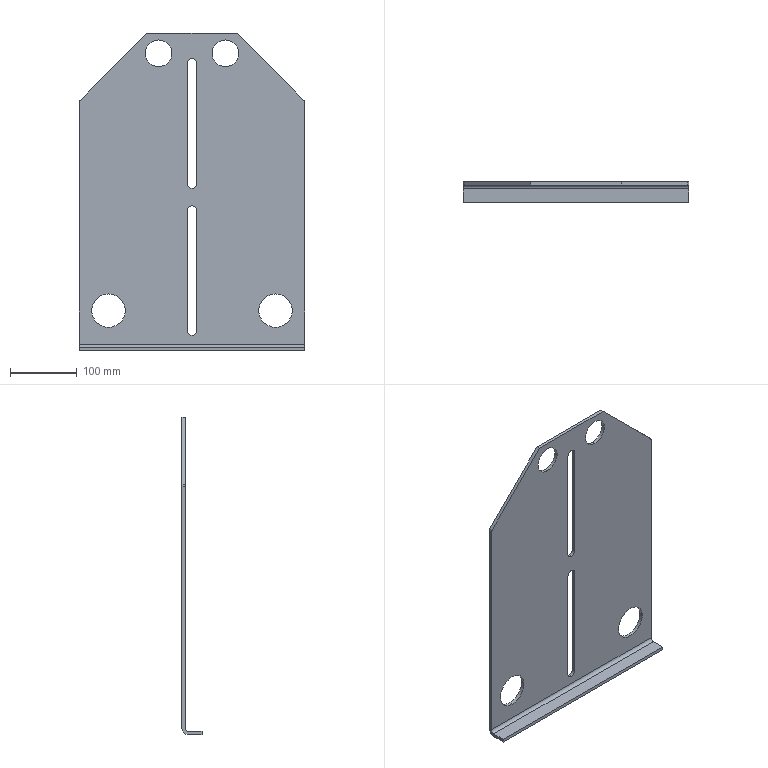Component | SolidWorks | 006TransformerBasePlate-1 | 1 solid | 32 faces | box 338 x 30 x 475 mm | volume 729103 mm3 | cylinder 18 | plane 14 | commonest cylinder face diameters 14 x6 50 x4 40 x4 10 x3 20 x1 | material Plain Carbon Steel
STEP:
#1=COLOUR_RGB('',0.7922,0.8196,0.9333);
#2=FILL_AREA_STYLE_COLOUR('',#1);
#3=FILL_AREA_STYLE('',(#2));
#4=SURFACE_STYLE_FILL_AREA(#3);
#5=SURFACE_SIDE_STYLE('',(#4));
#6=SURFACE_STYLE_USAGE(.BOTH.,#5);
#7=PRESENTATION_STYLE_ASSIGNMENT((#6));
#8=CARTESIAN_POINT('',(10.039,25.276,-15.591));
#9=VERTEX_POINT('',#8);
#10=CARTESIAN_POINT('',(10.039,25.276,-17.559));
#11=VERTEX_POINT('',#10);
#12=CARTESIAN_POINT('',(10.039,25.276,-16.575));
#13=DIRECTION('',(0.,1.,0.));
#14=DIRECTION('',(0.,0.,1.));
#15=AXIS2_PLACEMENT_3D('',#12,#13,#14);
#16=CIRCLE('',#15,0.9843);
#17=EDGE_CURVE('',#9,#11,#16,.T.);
#18=ORIENTED_EDGE('',*,*,#17,.F.);
#19=CARTESIAN_POINT('',(10.039,25.472,-15.591));
#20=VERTEX_POINT('',#19);
#21=CARTESIAN_POINT('',(10.039,24.291,-15.591));
#22=DIRECTION('',(0.,1.,0.));
#23=VECTOR('',#22,39.37);
#24=LINE('',#21,#23);
#25=EDGE_CURVE('',#9,#20,#24,.T.);
#26=ORIENTED_EDGE('',*,*,#25,.T.);
#27=CARTESIAN_POINT('',(10.039,25.472,-17.559));
#28=VERTEX_POINT('',#27);
#29=CARTESIAN_POINT('',(10.039,25.472,-16.575));
#30=DIRECTION('',(0.,1.,0.));
#31=DIRECTION('',(0.,0.,-1.));
#32=AXIS2_PLACEMENT_3D('',#29,#30,#31);
#33=CIRCLE('',#32,0.9843);
#34=EDGE_CURVE('',#20,#28,#33,.T.);
#35=ORIENTED_EDGE('',*,*,#34,.T.);
#36=CARTESIAN_POINT('',(10.039,24.291,-17.559));
#37=DIRECTION('',(0.,1.,0.));
#38=VECTOR('',#37,39.37);
#39=LINE('',#36,#38);
#40=EDGE_CURVE('',#11,#28,#39,.T.);
#41=ORIENTED_EDGE('',*,*,#40,.F.);
#42=EDGE_LOOP('',(#18,#26,#35,#41));
#43=FACE_OUTER_BOUND('',#42,.T.);
#44=CARTESIAN_POINT('',(10.039,24.291,-16.575));
#45=DIRECTION('',(0.,1.,0.));
#46=DIRECTION('',(0.,0.,-1.));
#47=AXIS2_PLACEMENT_3D('',#44,#45,#46);
#48=CYLINDRICAL_SURFACE('',#47,0.9843);
#49=ADVANCED_FACE('',(#43),#48,.F.);
#50=CARTESIAN_POINT('',(0.1969,25.276,-15.591));
#51=VERTEX_POINT('',#50);
#52=CARTESIAN_POINT('',(0.1969,25.276,-17.559));
#53=VERTEX_POINT('',#52);
#54=CARTESIAN_POINT('',(0.1969,25.276,-16.575));
#55=DIRECTION('',(0.,1.,0.));
#56=DIRECTION('',(0.,0.,1.));
#57=AXIS2_PLACEMENT_3D('',#54,#55,#56);
#58=CIRCLE('',#57,0.9843);
#59=EDGE_CURVE('',#51,#53,#58,.T.);
#60=ORIENTED_EDGE('',*,*,#59,.F.);
#61=CARTESIAN_POINT('',(0.1969,25.472,-15.591));
#62=VERTEX_POINT('',#61);
#63=CARTESIAN_POINT('',(0.1969,24.291,-15.591));
#64=DIRECTION('',(0.,1.,0.));
#65=VECTOR('',#64,39.37);
#66=LINE('',#63,#65);
#67=EDGE_CURVE('',#51,#62,#66,.T.);
#68=ORIENTED_EDGE('',*,*,#67,.T.);
#69=CARTESIAN_POINT('',(0.1969,25.472,-17.559));
#70=VERTEX_POINT('',#69);
#71=CARTESIAN_POINT('',(0.1969,25.472,-16.575));
#72=DIRECTION('',(0.,1.,0.));
#73=DIRECTION('',(0.,0.,-1.));
#74=AXIS2_PLACEMENT_3D('',#71,#72,#73);
#75=CIRCLE('',#74,0.9843);
#76=EDGE_CURVE('',#62,#70,#75,.T.);
#77=ORIENTED_EDGE('',*,*,#76,.T.);
#78=CARTESIAN_POINT('',(0.1969,24.291,-17.559));
#79=DIRECTION('',(0.,1.,0.));
#80=VECTOR('',#79,39.37);
#81=LINE('',#78,#80);
#82=EDGE_CURVE('',#53,#70,#81,.T.);
#83=ORIENTED_EDGE('',*,*,#82,.F.);
#84=EDGE_LOOP('',(#60,#68,#77,#83));
#85=FACE_OUTER_BOUND('',#84,.T.);
#86=CARTESIAN_POINT('',(0.1969,24.291,-16.575));
#87=DIRECTION('',(0.,1.,0.));
#88=DIRECTION('',(0.,0.,-1.));
#89=AXIS2_PLACEMENT_3D('',#86,#87,#88);
#90=CYLINDRICAL_SURFACE('',#89,0.9843);
#91=ADVANCED_FACE('',(#85),#90,.F.);
#92=CARTESIAN_POINT('',(7.087,25.276,-0.6299));
#93=VERTEX_POINT('',#92);
#94=CARTESIAN_POINT('',(7.087,25.276,-2.205));
#95=VERTEX_POINT('',#94);
#96=CARTESIAN_POINT('',(7.087,25.276,-1.417));
#97=DIRECTION('',(0.,1.,0.));
#98=DIRECTION('',(0.,0.,1.));
#99=AXIS2_PLACEMENT_3D('',#96,#97,#98);
#100=CIRCLE('',#99,0.7874);
#101=EDGE_CURVE('',#93,#95,#100,.T.);
#102=ORIENTED_EDGE('',*,*,#101,.F.);
#103=CARTESIAN_POINT('',(7.087,25.472,-0.6299));
#104=VERTEX_POINT('',#103);
#105=CARTESIAN_POINT('',(7.087,24.291,-0.6299));
#106=DIRECTION('',(0.,1.,0.));
#107=VECTOR('',#106,39.37);
#108=LINE('',#105,#107);
#109=EDGE_CURVE('',#93,#104,#108,.T.);
#110=ORIENTED_EDGE('',*,*,#109,.T.);
#111=CARTESIAN_POINT('',(7.087,25.472,-2.205));
#112=VERTEX_POINT('',#111);
#113=CARTESIAN_POINT('',(7.087,25.472,-1.417));
#114=DIRECTION('',(0.,1.,0.));
#115=DIRECTION('',(0.,0.,-1.));
#116=AXIS2_PLACEMENT_3D('',#113,#114,#115);
#117=CIRCLE('',#116,0.7874);
#118=EDGE_CURVE('',#104,#112,#117,.T.);
#119=ORIENTED_EDGE('',*,*,#118,.T.);
#120=CARTESIAN_POINT('',(7.087,24.291,-2.205));
#121=DIRECTION('',(0.,1.,0.));
#122=VECTOR('',#121,39.37);
#123=LINE('',#120,#122);
#124=EDGE_CURVE('',#95,#112,#123,.T.);
#125=ORIENTED_EDGE('',*,*,#124,.F.);
#126=EDGE_LOOP('',(#102,#110,#119,#125));
#127=FACE_OUTER_BOUND('',#126,.T.);
#128=CARTESIAN_POINT('',(7.087,24.291,-1.417));
#129=DIRECTION('',(0.,1.,0.));
#130=DIRECTION('',(0.,0.,-1.));
#131=AXIS2_PLACEMENT_3D('',#128,#129,#130);
#132=CYLINDRICAL_SURFACE('',#131,0.7874);
#133=ADVANCED_FACE('',(#127),#132,.F.);
#134=CARTESIAN_POINT('',(3.15,25.276,-0.6299));
#135=VERTEX_POINT('',#134);
#136=CARTESIAN_POINT('',(3.15,25.276,-2.205));
#137=VERTEX_POINT('',#136);
#138=CARTESIAN_POINT('',(3.15,25.276,-1.417));
#139=DIRECTION('',(0.,1.,0.));
#140=DIRECTION('',(0.,0.,1.));
#141=AXIS2_PLACEMENT_3D('',#138,#139,#140);
#142=CIRCLE('',#141,0.7874);
#143=EDGE_CURVE('',#135,#137,#142,.T.);
#144=ORIENTED_EDGE('',*,*,#143,.F.);
#145=CARTESIAN_POINT('',(3.15,25.472,-0.6299));
#146=VERTEX_POINT('',#145);
#147=CARTESIAN_POINT('',(3.15,24.291,-0.6299));
#148=DIRECTION('',(0.,1.,0.));
#149=VECTOR('',#148,39.37);
#150=LINE('',#147,#149);
#151=EDGE_CURVE('',#135,#146,#150,.T.);
#152=ORIENTED_EDGE('',*,*,#151,.T.);
#153=CARTESIAN_POINT('',(3.15,25.472,-2.205));
#154=VERTEX_POINT('',#153);
#155=CARTESIAN_POINT('',(3.15,25.472,-1.417));
#156=DIRECTION('',(0.,1.,0.));
#157=DIRECTION('',(0.,0.,-1.));
#158=AXIS2_PLACEMENT_3D('',#155,#156,#157);
#159=CIRCLE('',#158,0.7874);
#160=EDGE_CURVE('',#146,#154,#159,.T.);
#161=ORIENTED_EDGE('',*,*,#160,.T.);
#162=CARTESIAN_POINT('',(3.15,24.291,-2.205));
#163=DIRECTION('',(0.,1.,0.));
#164=VECTOR('',#163,39.37);
#165=LINE('',#162,#164);
#166=EDGE_CURVE('',#137,#154,#165,.T.);
#167=ORIENTED_EDGE('',*,*,#166,.F.);
#168=EDGE_LOOP('',(#144,#152,#161,#167));
#169=FACE_OUTER_BOUND('',#168,.T.);
#170=CARTESIAN_POINT('',(3.15,24.291,-1.417));
#171=DIRECTION('',(0.,1.,0.));
#172=DIRECTION('',(0.,0.,-1.));
#173=AXIS2_PLACEMENT_3D('',#170,#171,#172);
#174=CYLINDRICAL_SURFACE('',#173,0.7874);
#175=ADVANCED_FACE('',(#169),#174,.F.);
#176=CARTESIAN_POINT('',(5.118,25.276,-18.031));
#177=VERTEX_POINT('',#176);
#178=CARTESIAN_POINT('',(4.843,25.276,-17.756));
#179=VERTEX_POINT('',#178);
#180=CARTESIAN_POINT('',(5.118,25.276,-17.756));
#181=DIRECTION('',(0.,1.,0.));
#182=DIRECTION('',(0.,0.,1.));
#183=AXIS2_PLACEMENT_3D('',#180,#181,#182);
#184=CIRCLE('',#183,0.2756);
#185=EDGE_CURVE('',#177,#179,#184,.T.);
#186=ORIENTED_EDGE('',*,*,#185,.F.);
#187=CARTESIAN_POINT('',(5.118,25.472,-18.031));
#188=VERTEX_POINT('',#187);
#189=CARTESIAN_POINT('',(5.118,25.276,-18.031));
#190=DIRECTION('',(0.,1.,0.));
#191=VECTOR('',#190,39.37);
#192=LINE('',#189,#191);
#193=EDGE_CURVE('',#177,#188,#192,.T.);
#194=ORIENTED_EDGE('',*,*,#193,.T.);
#195=CARTESIAN_POINT('',(4.843,25.472,-17.756));
#196=VERTEX_POINT('',#195);
#197=CARTESIAN_POINT('',(5.118,25.472,-17.756));
#198=DIRECTION('',(0.,1.,0.));
#199=DIRECTION('',(0.,0.,-1.));
#200=AXIS2_PLACEMENT_3D('',#197,#198,#199);
#201=CIRCLE('',#200,0.2756);
#202=EDGE_CURVE('',#188,#196,#201,.T.);
#203=ORIENTED_EDGE('',*,*,#202,.T.);
#204=CARTESIAN_POINT('',(4.843,25.276,-17.756));
#205=DIRECTION('',(0.,1.,0.));
#206=VECTOR('',#205,39.37);
#207=LINE('',#204,#206);
#208=EDGE_CURVE('',#179,#196,#207,.T.);
#209=ORIENTED_EDGE('',*,*,#208,.F.);
#210=EDGE_LOOP('',(#186,#194,#203,#209));
#211=FACE_OUTER_BOUND('',#210,.T.);
#212=CARTESIAN_POINT('',(5.118,25.276,-17.756));
#213=DIRECTION('',(0.,1.,0.));
#214=DIRECTION('',(0.,0.,-1.));
#215=AXIS2_PLACEMENT_3D('',#212,#213,#214);
#216=CYLINDRICAL_SURFACE('',#215,0.2756);
#217=ADVANCED_FACE('',(#211),#216,.F.);
#218=CARTESIAN_POINT('',(5.118,25.276,-9.37));
#219=VERTEX_POINT('',#218);
#220=CARTESIAN_POINT('',(4.843,25.276,-9.094));
#221=VERTEX_POINT('',#220);
#222=CARTESIAN_POINT('',(5.118,25.276,-9.094));
#223=DIRECTION('',(0.,1.,0.));
#224=DIRECTION('',(0.,0.,1.));
#225=AXIS2_PLACEMENT_3D('',#222,#223,#224);
#226=CIRCLE('',#225,0.2756);
#227=EDGE_CURVE('',#219,#221,#226,.T.);
#228=ORIENTED_EDGE('',*,*,#227,.F.);
#229=CARTESIAN_POINT('',(5.118,25.472,-9.37));
#230=VERTEX_POINT('',#229);
#231=CARTESIAN_POINT('',(5.118,25.276,-9.37));
#232=DIRECTION('',(0.,1.,0.));
#233=VECTOR('',#232,39.37);
#234=LINE('',#231,#233);
#235=EDGE_CURVE('',#219,#230,#234,.T.);
#236=ORIENTED_EDGE('',*,*,#235,.T.);
#237=CARTESIAN_POINT('',(4.843,25.472,-9.094));
#238=VERTEX_POINT('',#237);
#239=CARTESIAN_POINT('',(5.118,25.472,-9.094));
#240=DIRECTION('',(0.,1.,0.));
#241=DIRECTION('',(0.,0.,-1.));
#242=AXIS2_PLACEMENT_3D('',#239,#240,#241);
#243=CIRCLE('',#242,0.2756);
#244=EDGE_CURVE('',#230,#238,#243,.T.);
#245=ORIENTED_EDGE('',*,*,#244,.T.);
#246=CARTESIAN_POINT('',(4.843,25.276,-9.094));
#247=DIRECTION('',(0.,1.,0.));
#248=VECTOR('',#247,39.37);
#249=LINE('',#246,#248);
#250=EDGE_CURVE('',#221,#238,#249,.T.);
#251=ORIENTED_EDGE('',*,*,#250,.F.);
#252=EDGE_LOOP('',(#228,#236,#245,#251));
#253=FACE_OUTER_BOUND('',#252,.T.);
#254=CARTESIAN_POINT('',(5.118,25.276,-9.094));
#255=DIRECTION('',(0.,1.,0.));
#256=DIRECTION('',(0.,0.,-1.));
#257=AXIS2_PLACEMENT_3D('',#254,#255,#256);
#258=CYLINDRICAL_SURFACE('',#257,0.2756);
#259=ADVANCED_FACE('',(#253),#258,.F.);
#260=CARTESIAN_POINT('',(10.039,25.276,-16.575));
#261=DIRECTION('',(0.,1.,0.));
#262=DIRECTION('',(0.,0.,1.));
#263=AXIS2_PLACEMENT_3D('',#260,#261,#262);
#264=CIRCLE('',#263,0.9843);
#265=EDGE_CURVE('',#11,#9,#264,.T.);
#266=ORIENTED_EDGE('',*,*,#265,.T.);
#267=ORIENTED_EDGE('',*,*,#17,.T.);
#268=EDGE_LOOP('',(#266,#267));
#269=FACE_BOUND('',#268,.T.);
#270=CARTESIAN_POINT('',(0.1969,25.276,-16.575));
#271=DIRECTION('',(0.,1.,0.));
#272=DIRECTION('',(0.,0.,1.));
#273=AXIS2_PLACEMENT_3D('',#270,#271,#272);
#274=CIRCLE('',#273,0.9843);
#275=EDGE_CURVE('',#53,#51,#274,.T.);
#276=ORIENTED_EDGE('',*,*,#275,.T.);
#277=ORIENTED_EDGE('',*,*,#59,.T.);
#278=EDGE_LOOP('',(#276,#277));
#279=FACE_BOUND('',#278,.T.);
#280=CARTESIAN_POINT('',(7.087,25.276,-1.417));
#281=DIRECTION('',(0.,1.,0.));
#282=DIRECTION('',(0.,0.,1.));
#283=AXIS2_PLACEMENT_3D('',#280,#281,#282);
#284=CIRCLE('',#283,0.7874);
#285=EDGE_CURVE('',#95,#93,#284,.T.);
#286=ORIENTED_EDGE('',*,*,#285,.T.);
#287=ORIENTED_EDGE('',*,*,#101,.T.);
#288=EDGE_LOOP('',(#286,#287));
#289=FACE_BOUND('',#288,.T.);
#290=CARTESIAN_POINT('',(3.15,25.276,-1.417));
#291=DIRECTION('',(0.,1.,0.));
#292=DIRECTION('',(0.,0.,1.));
#293=AXIS2_PLACEMENT_3D('',#290,#291,#292);
#294=CIRCLE('',#293,0.7874);
#295=EDGE_CURVE('',#137,#135,#294,.T.);
#296=ORIENTED_EDGE('',*,*,#295,.T.);
#297=ORIENTED_EDGE('',*,*,#143,.T.);
#298=EDGE_LOOP('',(#296,#297));
#299=FACE_BOUND('',#298,.T.);
#300=CARTESIAN_POINT('',(4.843,25.276,-10.669));
#301=VERTEX_POINT('',#300);
#302=CARTESIAN_POINT('',(5.394,25.276,-10.669));
#303=VERTEX_POINT('',#302);
#304=CARTESIAN_POINT('',(5.118,25.276,-10.669));
#305=DIRECTION('',(0.,1.,0.));
#306=DIRECTION('',(0.,0.,1.));
#307=AXIS2_PLACEMENT_3D('',#304,#305,#306);
#308=CIRCLE('',#307,0.2756);
#309=EDGE_CURVE('',#301,#303,#308,.T.);
#310=ORIENTED_EDGE('',*,*,#309,.T.);
#311=CARTESIAN_POINT('',(5.394,25.276,-17.756));
#312=VERTEX_POINT('',#311);
#313=CARTESIAN_POINT('',(5.394,25.276,-10.669));
#314=DIRECTION('',(0.,0.,-1.));
#315=VECTOR('',#314,39.37);
#316=LINE('',#313,#315);
#317=EDGE_CURVE('',#303,#312,#316,.T.);
#318=ORIENTED_EDGE('',*,*,#317,.T.);
#319=CARTESIAN_POINT('',(5.118,25.276,-17.756));
#320=DIRECTION('',(0.,1.,0.));
#321=DIRECTION('',(0.,0.,1.));
#322=AXIS2_PLACEMENT_3D('',#319,#320,#321);
#323=CIRCLE('',#322,0.2756);
#324=EDGE_CURVE('',#312,#177,#323,.T.);
#325=ORIENTED_EDGE('',*,*,#324,.T.);
#326=ORIENTED_EDGE('',*,*,#185,.T.);
#327=CARTESIAN_POINT('',(4.843,25.276,-10.669));
#328=DIRECTION('',(-0.,0.,1.));
#329=VECTOR('',#328,39.37);
#330=LINE('',#327,#329);
#331=EDGE_CURVE('',#179,#301,#330,.T.);
#332=ORIENTED_EDGE('',*,*,#331,.T.);
#333=EDGE_LOOP('',(#310,#318,#325,#326,#332));
#334=FACE_BOUND('',#333,.T.);
#335=CARTESIAN_POINT('',(4.843,25.276,-2.008));
#336=VERTEX_POINT('',#335);
#337=CARTESIAN_POINT('',(5.394,25.276,-2.008));
#338=VERTEX_POINT('',#337);
#339=CARTESIAN_POINT('',(5.118,25.276,-2.008));
#340=DIRECTION('',(0.,1.,0.));
#341=DIRECTION('',(0.,0.,1.));
#342=AXIS2_PLACEMENT_3D('',#339,#340,#341);
#343=CIRCLE('',#342,0.2756);
#344=EDGE_CURVE('',#336,#338,#343,.T.);
#345=ORIENTED_EDGE('',*,*,#344,.T.);
#346=CARTESIAN_POINT('',(5.394,25.276,-9.094));
#347=VERTEX_POINT('',#346);
#348=CARTESIAN_POINT('',(5.394,25.276,-2.008));
#349=DIRECTION('',(0.,0.,-1.));
#350=VECTOR('',#349,39.37);
#351=LINE('',#348,#350);
#352=EDGE_CURVE('',#338,#347,#351,.T.);
#353=ORIENTED_EDGE('',*,*,#352,.T.);
#354=CARTESIAN_POINT('',(5.118,25.276,-9.094));
#355=DIRECTION('',(0.,1.,0.));
#356=DIRECTION('',(0.,0.,1.));
#357=AXIS2_PLACEMENT_3D('',#354,#355,#356);
#358=CIRCLE('',#357,0.2756);
#359=EDGE_CURVE('',#347,#219,#358,.T.);
#360=ORIENTED_EDGE('',*,*,#359,.T.);
#361=ORIENTED_EDGE('',*,*,#227,.T.);
#362=CARTESIAN_POINT('',(4.843,25.276,-2.008));
#363=DIRECTION('',(0.,0.,1.));
#364=VECTOR('',#363,39.37);
#365=LINE('',#362,#364);
#366=EDGE_CURVE('',#221,#336,#365,.T.);
#367=ORIENTED_EDGE('',*,*,#366,.T.);
#368=EDGE_LOOP('',(#345,#353,#360,#361,#367));
#369=FACE_BOUND('',#368,.T.);
#370=CARTESIAN_POINT('',(-1.535,25.276,-18.543));
#371=VERTEX_POINT('',#370);
#372=CARTESIAN_POINT('',(-1.535,25.276,-4.314));
#373=VERTEX_POINT('',#372);
#374=CARTESIAN_POINT('',(-1.535,25.276,-4.232));
#375=DIRECTION('',(-0.,0.,1.));
#376=VECTOR('',#375,39.37);
#377=LINE('',#374,#376);
#378=EDGE_CURVE('',#371,#373,#377,.T.);
#379=ORIENTED_EDGE('',*,*,#378,.F.);
#380=CARTESIAN_POINT('',(11.772,25.276,-18.543));
#381=VERTEX_POINT('',#380);
#382=CARTESIAN_POINT('',(11.772,25.276,-18.543));
#383=DIRECTION('',(1.,0.,0.));
#384=VECTOR('',#383,39.37);
#385=LINE('',#382,#384);
#386=EDGE_CURVE('',#371,#381,#385,.T.);
#387=ORIENTED_EDGE('',*,*,#386,.T.);
#388=CARTESIAN_POINT('',(11.772,25.276,-4.314));
#389=VERTEX_POINT('',#388);
#390=CARTESIAN_POINT('',(11.772,25.276,-4.232));
#391=DIRECTION('',(-0.,0.,-1.));
#392=VECTOR('',#391,39.37);
#393=LINE('',#390,#392);
#394=EDGE_CURVE('',#389,#381,#393,.T.);
#395=ORIENTED_EDGE('',*,*,#394,.F.);
#396=CARTESIAN_POINT('',(11.714,25.276,-4.175));
#397=VERTEX_POINT('',#396);
#398=CARTESIAN_POINT('',(11.575,25.276,-4.314));
#399=DIRECTION('',(0.,-1.,0.));
#400=DIRECTION('',(0.,0.,1.));
#401=AXIS2_PLACEMENT_3D('',#398,#399,#400);
#402=CIRCLE('',#401,0.1969);
#403=EDGE_CURVE('',#389,#397,#402,.T.);
#404=ORIENTED_EDGE('',*,*,#403,.T.);
#405=CARTESIAN_POINT('',(7.776,25.276,-0.2362));
#406=VERTEX_POINT('',#405);
#407=CARTESIAN_POINT('',(11.772,25.276,-4.232));
#408=DIRECTION('',(0.7071,0.,-0.7071));
#409=VECTOR('',#408,39.37);
#410=LINE('',#407,#409);
#411=EDGE_CURVE('',#406,#397,#410,.T.);
#412=ORIENTED_EDGE('',*,*,#411,.F.);
#413=CARTESIAN_POINT('',(2.461,25.276,-0.2362));
#414=VERTEX_POINT('',#413);
#415=CARTESIAN_POINT('',(7.776,25.276,-0.2362));
#416=DIRECTION('',(1.,0.,0.));
#417=VECTOR('',#416,39.37);
#418=LINE('',#415,#417);
#419=EDGE_CURVE('',#414,#406,#418,.T.);
#420=ORIENTED_EDGE('',*,*,#419,.F.);
#421=CARTESIAN_POINT('',(-1.478,25.276,-4.175));
#422=VERTEX_POINT('',#421);
#423=CARTESIAN_POINT('',(-1.535,25.276,-4.232));
#424=DIRECTION('',(0.7071,0.,0.7071));
#425=VECTOR('',#424,39.37);
#426=LINE('',#423,#425);
#427=EDGE_CURVE('',#422,#414,#426,.T.);
#428=ORIENTED_EDGE('',*,*,#427,.F.);
#429=CARTESIAN_POINT('',(-1.339,25.276,-4.314));
#430=DIRECTION('',(0.,-1.,0.));
#431=DIRECTION('',(0.,0.,1.));
#432=AXIS2_PLACEMENT_3D('',#429,#430,#431);
#433=CIRCLE('',#432,0.1969);
#434=EDGE_CURVE('',#422,#373,#433,.T.);
#435=ORIENTED_EDGE('',*,*,#434,.T.);
#436=EDGE_LOOP('',(#379,#387,#395,#404,#412,#420,#428,#435));
#437=FACE_OUTER_BOUND('',#436,.T.);
#438=CARTESIAN_POINT('',(-1.535,25.276,-18.937));
#439=DIRECTION('',(0.,-1.,0.));
#440=DIRECTION('',(0.,0.,1.));
#441=AXIS2_PLACEMENT_3D('',#438,#439,#440);
#442=PLANE('',#441);
#443=ADVANCED_FACE('',(#269,#279,#289,#299,#334,#369,#437),#442,.T.);
#444=CARTESIAN_POINT('',(-1.535,25.079,-18.937));
#445=VERTEX_POINT('',#444);
#446=CARTESIAN_POINT('',(-1.535,24.291,-18.937));
#447=VERTEX_POINT('',#446);
#448=CARTESIAN_POINT('',(-1.535,25.472,-18.937));
#449=DIRECTION('',(0.,-1.,0.));
#450=VECTOR('',#449,39.37);
#451=LINE('',#448,#450);
#452=EDGE_CURVE('',#445,#447,#451,.T.);
#453=ORIENTED_EDGE('',*,*,#452,.F.);
#454=CARTESIAN_POINT('',(11.772,25.079,-18.937));
#455=VERTEX_POINT('',#454);
#456=CARTESIAN_POINT('',(11.772,25.079,-18.937));
#457=DIRECTION('',(1.,0.,0.));
#458=VECTOR('',#457,39.37);
#459=LINE('',#456,#458);
#460=EDGE_CURVE('',#445,#455,#459,.T.);
#461=ORIENTED_EDGE('',*,*,#460,.T.);
#462=CARTESIAN_POINT('',(11.772,24.291,-18.937));
#463=VERTEX_POINT('',#462);
#464=CARTESIAN_POINT('',(11.772,25.472,-18.937));
#465=DIRECTION('',(0.,-1.,0.));
#466=VECTOR('',#465,39.37);
#467=LINE('',#464,#466);
#468=EDGE_CURVE('',#455,#463,#467,.T.);
#469=ORIENTED_EDGE('',*,*,#468,.T.);
#470=CARTESIAN_POINT('',(-2.539,24.291,-18.937));
#471=DIRECTION('',(1.,0.,0.));
#472=VECTOR('',#471,39.37);
#473=LINE('',#470,#472);
#474=EDGE_CURVE('',#447,#463,#473,.T.);
#475=ORIENTED_EDGE('',*,*,#474,.F.);
#476=EDGE_LOOP('',(#453,#461,#469,#475));
#477=FACE_OUTER_BOUND('',#476,.T.);
#478=CARTESIAN_POINT('',(11.772,25.472,-18.937));
#479=DIRECTION('',(0.,0.,1.));
#480=DIRECTION('',(0.,1.,0.));
#481=AXIS2_PLACEMENT_3D('',#478,#479,#480);
#482=PLANE('',#481);
#483=ADVANCED_FACE('',(#477),#482,.F.);
#484=CARTESIAN_POINT('',(-1.535,25.472,-18.543));
#485=VERTEX_POINT('',#484);
#486=CARTESIAN_POINT('',(-1.535,25.472,-4.314));
#487=VERTEX_POINT('',#486);
#488=CARTESIAN_POINT('',(-1.535,25.472,-4.232));
#489=DIRECTION('',(-0.,0.,1.));
#490=VECTOR('',#489,39.37);
#491=LINE('',#488,#490);
#492=EDGE_CURVE('',#485,#487,#491,.T.);
#493=ORIENTED_EDGE('',*,*,#492,.F.);
#494=CARTESIAN_POINT('',(-1.535,25.079,-18.543));
#495=DIRECTION('',(-1.,0.,-0.));
#496=DIRECTION('',(0.,0.,-1.));
#497=AXIS2_PLACEMENT_3D('',#494,#495,#496);
#498=CIRCLE('',#497,0.3937);
#499=EDGE_CURVE('',#485,#445,#498,.T.);
#500=ORIENTED_EDGE('',*,*,#499,.T.);
#501=ORIENTED_EDGE('',*,*,#452,.T.);
#502=CARTESIAN_POINT('',(-1.535,24.291,-18.74));
#503=VERTEX_POINT('',#502);
#504=CARTESIAN_POINT('',(-1.535,24.291,-18.74));
#505=DIRECTION('',(-0.,0.,1.));
#506=VECTOR('',#505,39.37);
#507=LINE('',#504,#506);
#508=EDGE_CURVE('',#447,#503,#507,.T.);
#509=ORIENTED_EDGE('',*,*,#508,.T.);
#510=CARTESIAN_POINT('',(-1.535,25.079,-18.74));
#511=VERTEX_POINT('',#510);
#512=CARTESIAN_POINT('',(-1.535,25.276,-18.74));
#513=DIRECTION('',(-0.,1.,0.));
#514=VECTOR('',#513,39.37);
#515=LINE('',#512,#514);
#516=EDGE_CURVE('',#503,#511,#515,.T.);
#517=ORIENTED_EDGE('',*,*,#516,.T.);
#518=CARTESIAN_POINT('',(-1.535,25.079,-18.543));
#519=DIRECTION('',(1.,0.,0.));
#520=DIRECTION('',(0.,0.,-1.));
#521=AXIS2_PLACEMENT_3D('',#518,#519,#520);
#522=CIRCLE('',#521,0.1969);
#523=EDGE_CURVE('',#511,#371,#522,.T.);
#524=ORIENTED_EDGE('',*,*,#523,.T.);
#525=ORIENTED_EDGE('',*,*,#378,.T.);
#526=CARTESIAN_POINT('',(-1.535,25.472,-4.314));
#527=DIRECTION('',(0.,1.,0.));
#528=VECTOR('',#527,39.37);
#529=LINE('',#526,#528);
#530=EDGE_CURVE('',#373,#487,#529,.T.);
#531=ORIENTED_EDGE('',*,*,#530,.T.);
#532=EDGE_LOOP('',(#493,#500,#501,#509,#517,#524,#525,#531));
#533=FACE_OUTER_BOUND('',#532,.T.);
#534=CARTESIAN_POINT('',(-1.535,25.472,-4.232));
#535=DIRECTION('',(1.,0.,0.));
#536=DIRECTION('',(0.,0.,-1.));
#537=AXIS2_PLACEMENT_3D('',#534,#535,#536);
#538=PLANE('',#537);
#539=ADVANCED_FACE('',(#533),#538,.F.);
#540=CARTESIAN_POINT('',(-1.478,25.472,-4.175));
#541=VERTEX_POINT('',#540);
#542=CARTESIAN_POINT('',(2.461,25.472,-0.2362));
#543=VERTEX_POINT('',#542);
#544=CARTESIAN_POINT('',(-1.535,25.472,-4.232));
#545=DIRECTION('',(0.7071,0.,0.7071));
#546=VECTOR('',#545,39.37);
#547=LINE('',#544,#546);
#548=EDGE_CURVE('',#541,#543,#547,.T.);
#549=ORIENTED_EDGE('',*,*,#548,.F.);
#550=CARTESIAN_POINT('',(-1.478,25.472,-4.175));
#551=DIRECTION('',(0.,-1.,0.));
#552=VECTOR('',#551,39.37);
#553=LINE('',#550,#552);
#554=EDGE_CURVE('',#541,#422,#553,.T.);
#555=ORIENTED_EDGE('',*,*,#554,.T.);
#556=ORIENTED_EDGE('',*,*,#427,.T.);
#557=CARTESIAN_POINT('',(2.461,25.472,-0.2362));
#558=DIRECTION('',(0.,-1.,0.));
#559=VECTOR('',#558,39.37);
#560=LINE('',#557,#559);
#561=EDGE_CURVE('',#543,#414,#560,.T.);
#562=ORIENTED_EDGE('',*,*,#561,.F.);
#563=EDGE_LOOP('',(#549,#555,#556,#562));
#564=FACE_OUTER_BOUND('',#563,.T.);
#565=CARTESIAN_POINT('',(-1.535,25.472,-4.232));
#566=DIRECTION('',(0.7071,0.,-0.7071));
#567=DIRECTION('',(-0.7071,0.,-0.7071));
#568=AXIS2_PLACEMENT_3D('',#565,#566,#567);
#569=PLANE('',#568);
#570=ADVANCED_FACE('',(#564),#569,.F.);
#571=ORIENTED_EDGE('',*,*,#419,.T.);
#572=CARTESIAN_POINT('',(7.776,25.472,-0.2362));
#573=VERTEX_POINT('',#572);
#574=CARTESIAN_POINT('',(7.776,25.472,-0.2362));
#575=DIRECTION('',(0.,-1.,0.));
#576=VECTOR('',#575,39.37);
#577=LINE('',#574,#576);
#578=EDGE_CURVE('',#573,#406,#577,.T.);
#579=ORIENTED_EDGE('',*,*,#578,.F.);
#580=CARTESIAN_POINT('',(7.776,25.472,-0.2362));
#581=DIRECTION('',(1.,0.,0.));
#582=VECTOR('',#581,39.37);
#583=LINE('',#580,#582);
#584=EDGE_CURVE('',#543,#573,#583,.T.);
#585=ORIENTED_EDGE('',*,*,#584,.F.);
#586=ORIENTED_EDGE('',*,*,#561,.T.);
#587=EDGE_LOOP('',(#571,#579,#585,#586));
#588=FACE_OUTER_BOUND('',#587,.T.);
#589=CARTESIAN_POINT('',(7.776,25.472,-0.2362));
#590=DIRECTION('',(0.,0.,-1.));
#591=DIRECTION('',(0.,-1.,0.));
#592=AXIS2_PLACEMENT_3D('',#589,#590,#591);
#593=PLANE('',#592);
#594=ADVANCED_FACE('',(#588),#593,.F.);
#595=ORIENTED_EDGE('',*,*,#411,.T.);
#596=CARTESIAN_POINT('',(11.714,25.472,-4.175));
#597=VERTEX_POINT('',#596);
#598=CARTESIAN_POINT('',(11.714,25.472,-4.175));
#599=DIRECTION('',(0.,1.,0.));
#600=VECTOR('',#599,39.37);
#601=LINE('',#598,#600);
#602=EDGE_CURVE('',#397,#597,#601,.T.);
#603=ORIENTED_EDGE('',*,*,#602,.T.);
#604=CARTESIAN_POINT('',(11.772,25.472,-4.232));
#605=DIRECTION('',(0.7071,0.,-0.7071));
#606=VECTOR('',#605,39.37);
#607=LINE('',#604,#606);
#608=EDGE_CURVE('',#573,#597,#607,.T.);
#609=ORIENTED_EDGE('',*,*,#608,.F.);
#610=ORIENTED_EDGE('',*,*,#578,.T.);
#611=EDGE_LOOP('',(#595,#603,#609,#610));
#612=FACE_OUTER_BOUND('',#611,.T.);
#613=CARTESIAN_POINT('',(11.772,25.472,-4.232));
#614=DIRECTION('',(-0.7071,0.,-0.7071));
#615=DIRECTION('',(-0.7071,0.,0.7071));
#616=AXIS2_PLACEMENT_3D('',#613,#614,#615);
#617=PLANE('',#616);
#618=ADVANCED_FACE('',(#612),#617,.F.);
#619=ORIENTED_EDGE('',*,*,#468,.F.);
#620=CARTESIAN_POINT('',(11.772,25.472,-18.543));
#621=VERTEX_POINT('',#620);
#622=CARTESIAN_POINT('',(11.772,25.079,-18.543));
#623=DIRECTION('',(1.,0.,-0.));
#624=DIRECTION('',(0.,0.,1.));
#625=AXIS2_PLACEMENT_3D('',#622,#623,#624);
#626=CIRCLE('',#625,0.3937);
#627=EDGE_CURVE('',#455,#621,#626,.T.);
#628=ORIENTED_EDGE('',*,*,#627,.T.);
#629=CARTESIAN_POINT('',(11.772,25.472,-4.314));
#630=VERTEX_POINT('',#629);
#631=CARTESIAN_POINT('',(11.772,25.472,-4.232));
#632=DIRECTION('',(-0.,0.,-1.));
#633=VECTOR('',#632,39.37);
#634=LINE('',#631,#633);
#635=EDGE_CURVE('',#630,#621,#634,.T.);
#636=ORIENTED_EDGE('',*,*,#635,.F.);
#637=CARTESIAN_POINT('',(11.772,25.472,-4.314));
#638=DIRECTION('',(0.,-1.,0.));
#639=VECTOR('',#638,39.37);
#640=LINE('',#637,#639);
#641=EDGE_CURVE('',#630,#389,#640,.T.);
#642=ORIENTED_EDGE('',*,*,#641,.T.);
#643=ORIENTED_EDGE('',*,*,#394,.T.);
#644=CARTESIAN_POINT('',(11.772,25.079,-18.74));
#645=VERTEX_POINT('',#644);
#646=CARTESIAN_POINT('',(11.772,25.079,-18.543));
#647=DIRECTION('',(-1.,0.,0.));
#648=DIRECTION('',(0.,0.,1.));
#649=AXIS2_PLACEMENT_3D('',#646,#647,#648);
#650=CIRCLE('',#649,0.1969);
#651=EDGE_CURVE('',#381,#645,#650,.T.);
#652=ORIENTED_EDGE('',*,*,#651,.T.);
#653=CARTESIAN_POINT('',(11.772,24.291,-18.74));
#654=VERTEX_POINT('',#653);
#655=CARTESIAN_POINT('',(11.772,25.276,-18.74));
#656=DIRECTION('',(0.,-1.,-0.));
#657=VECTOR('',#656,39.37);
#658=LINE('',#655,#657);
#659=EDGE_CURVE('',#645,#654,#658,.T.);
#660=ORIENTED_EDGE('',*,*,#659,.T.);
#661=CARTESIAN_POINT('',(11.772,24.291,-18.74));
#662=DIRECTION('',(0.,0.,-1.));
#663=VECTOR('',#662,39.37);
#664=LINE('',#661,#663);
#665=EDGE_CURVE('',#654,#463,#664,.T.);
#666=ORIENTED_EDGE('',*,*,#665,.T.);
#667=EDGE_LOOP('',(#619,#628,#636,#642,#643,#652,#660,#666));
#668=FACE_OUTER_BOUND('',#667,.T.);
#669=CARTESIAN_POINT('',(11.772,25.472,-4.232));
#670=DIRECTION('',(-1.,0.,0.));
#671=DIRECTION('',(0.,0.,1.));
#672=AXIS2_PLACEMENT_3D('',#669,#670,#671);
#673=PLANE('',#672);
#674=ADVANCED_FACE('',(#668),#673,.F.);
#675=CARTESIAN_POINT('',(10.039,25.472,-16.575));
#676=DIRECTION('',(0.,1.,0.));
#677=DIRECTION('',(0.,0.,-1.));
#678=AXIS2_PLACEMENT_3D('',#675,#676,#677);
#679=CIRCLE('',#678,0.9843);
#680=EDGE_CURVE('',#28,#20,#679,.T.);
#681=ORIENTED_EDGE('',*,*,#680,.F.);
#682=ORIENTED_EDGE('',*,*,#34,.F.);
#683=EDGE_LOOP('',(#681,#682));
#684=FACE_BOUND('',#683,.T.);
#685=CARTESIAN_POINT('',(0.1969,25.472,-16.575));
#686=DIRECTION('',(0.,1.,0.));
#687=DIRECTION('',(0.,0.,-1.));
#688=AXIS2_PLACEMENT_3D('',#685,#686,#687);
#689=CIRCLE('',#688,0.9843);
#690=EDGE_CURVE('',#70,#62,#689,.T.);
#691=ORIENTED_EDGE('',*,*,#690,.F.);
#692=ORIENTED_EDGE('',*,*,#76,.F.);
#693=EDGE_LOOP('',(#691,#692));
#694=FACE_BOUND('',#693,.T.);
#695=CARTESIAN_POINT('',(7.087,25.472,-1.417));
#696=DIRECTION('',(0.,1.,0.));
#697=DIRECTION('',(0.,0.,-1.));
#698=AXIS2_PLACEMENT_3D('',#695,#696,#697);
#699=CIRCLE('',#698,0.7874);
#700=EDGE_CURVE('',#112,#104,#699,.T.);
#701=ORIENTED_EDGE('',*,*,#700,.F.);
#702=ORIENTED_EDGE('',*,*,#118,.F.);
#703=EDGE_LOOP('',(#701,#702));
#704=FACE_BOUND('',#703,.T.);
#705=CARTESIAN_POINT('',(3.15,25.472,-1.417));
#706=DIRECTION('',(0.,1.,0.));
#707=DIRECTION('',(0.,0.,-1.));
#708=AXIS2_PLACEMENT_3D('',#705,#706,#707);
#709=CIRCLE('',#708,0.7874);
#710=EDGE_CURVE('',#154,#146,#709,.T.);
#711=ORIENTED_EDGE('',*,*,#710,.F.);
#712=ORIENTED_EDGE('',*,*,#160,.F.);
#713=EDGE_LOOP('',(#711,#712));
#714=FACE_BOUND('',#713,.T.);
#715=CARTESIAN_POINT('',(5.394,25.472,-10.669));
#716=VERTEX_POINT('',#715);
#717=CARTESIAN_POINT('',(5.394,25.472,-17.756));
#718=VERTEX_POINT('',#717);
#719=CARTESIAN_POINT('',(5.394,25.472,-10.669));
#720=DIRECTION('',(0.,0.,-1.));
#721=VECTOR('',#720,39.37);
#722=LINE('',#719,#721);
#723=EDGE_CURVE('',#716,#718,#722,.T.);
#724=ORIENTED_EDGE('',*,*,#723,.F.);
#725=CARTESIAN_POINT('',(4.843,25.472,-10.669));
#726=VERTEX_POINT('',#725);
#727=CARTESIAN_POINT('',(5.118,25.472,-10.669));
#728=DIRECTION('',(0.,1.,0.));
#729=DIRECTION('',(0.,0.,-1.));
#730=AXIS2_PLACEMENT_3D('',#727,#728,#729);
#731=CIRCLE('',#730,0.2756);
#732=EDGE_CURVE('',#726,#716,#731,.T.);
#733=ORIENTED_EDGE('',*,*,#732,.F.);
#734=CARTESIAN_POINT('',(4.843,25.472,-10.669));
#735=DIRECTION('',(-0.,0.,1.));
#736=VECTOR('',#735,39.37);
#737=LINE('',#734,#736);
#738=EDGE_CURVE('',#196,#726,#737,.T.);
#739=ORIENTED_EDGE('',*,*,#738,.F.);
#740=ORIENTED_EDGE('',*,*,#202,.F.);
#741=CARTESIAN_POINT('',(5.118,25.472,-17.756));
#742=DIRECTION('',(0.,1.,0.));
#743=DIRECTION('',(0.,0.,-1.));
#744=AXIS2_PLACEMENT_3D('',#741,#742,#743);
#745=CIRCLE('',#744,0.2756);
#746=EDGE_CURVE('',#718,#188,#745,.T.);
#747=ORIENTED_EDGE('',*,*,#746,.F.);
#748=EDGE_LOOP('',(#724,#733,#739,#740,#747));
#749=FACE_BOUND('',#748,.T.);
#750=CARTESIAN_POINT('',(5.394,25.472,-2.008));
#751=VERTEX_POINT('',#750);
#752=CARTESIAN_POINT('',(5.394,25.472,-9.094));
#753=VERTEX_POINT('',#752);
#754=CARTESIAN_POINT('',(5.394,25.472,-2.008));
#755=DIRECTION('',(0.,0.,-1.));
#756=VECTOR('',#755,39.37);
#757=LINE('',#754,#756);
#758=EDGE_CURVE('',#751,#753,#757,.T.);
#759=ORIENTED_EDGE('',*,*,#758,.F.);
#760=CARTESIAN_POINT('',(4.843,25.472,-2.008));
#761=VERTEX_POINT('',#760);
#762=CARTESIAN_POINT('',(5.118,25.472,-2.008));
#763=DIRECTION('',(0.,1.,0.));
#764=DIRECTION('',(0.,0.,-1.));
#765=AXIS2_PLACEMENT_3D('',#762,#763,#764);
#766=CIRCLE('',#765,0.2756);
#767=EDGE_CURVE('',#761,#751,#766,.T.);
#768=ORIENTED_EDGE('',*,*,#767,.F.);
#769=CARTESIAN_POINT('',(4.843,25.472,-2.008));
#770=DIRECTION('',(0.,0.,1.));
#771=VECTOR('',#770,39.37);
#772=LINE('',#769,#771);
#773=EDGE_CURVE('',#238,#761,#772,.T.);
#774=ORIENTED_EDGE('',*,*,#773,.F.);
#775=ORIENTED_EDGE('',*,*,#244,.F.);
#776=CARTESIAN_POINT('',(5.118,25.472,-9.094));
#777=DIRECTION('',(0.,1.,0.));
#778=DIRECTION('',(0.,0.,-1.));
#779=AXIS2_PLACEMENT_3D('',#776,#777,#778);
#780=CIRCLE('',#779,0.2756);
#781=EDGE_CURVE('',#753,#230,#780,.T.);
#782=ORIENTED_EDGE('',*,*,#781,.F.);
#783=EDGE_LOOP('',(#759,#768,#774,#775,#782));
#784=FACE_BOUND('',#783,.T.);
#785=ORIENTED_EDGE('',*,*,#635,.T.);
#786=CARTESIAN_POINT('',(-1.535,25.472,-18.543));
#787=DIRECTION('',(-1.,0.,0.));
#788=VECTOR('',#787,39.37);
#789=LINE('',#786,#788);
#790=EDGE_CURVE('',#621,#485,#789,.T.);
#791=ORIENTED_EDGE('',*,*,#790,.T.);
#792=ORIENTED_EDGE('',*,*,#492,.T.);
#793=CARTESIAN_POINT('',(-1.339,25.472,-4.314));
#794=DIRECTION('',(0.,1.,0.));
#795=DIRECTION('',(-0.,0.,1.));
#796=AXIS2_PLACEMENT_3D('',#793,#794,#795);
#797=CIRCLE('',#796,0.1969);
#798=EDGE_CURVE('',#487,#541,#797,.T.);
#799=ORIENTED_EDGE('',*,*,#798,.T.);
#800=ORIENTED_EDGE('',*,*,#548,.T.);
#801=ORIENTED_EDGE('',*,*,#584,.T.);
#802=ORIENTED_EDGE('',*,*,#608,.T.);
#803=CARTESIAN_POINT('',(11.575,25.472,-4.314));
#804=DIRECTION('',(0.,1.,0.));
#805=DIRECTION('',(0.,0.,1.));
#806=AXIS2_PLACEMENT_3D('',#803,#804,#805);
#807=CIRCLE('',#806,0.1969);
#808=EDGE_CURVE('',#597,#630,#807,.T.);
#809=ORIENTED_EDGE('',*,*,#808,.T.);
#810=EDGE_LOOP('',(#785,#791,#792,#799,#800,#801,#802,#809));
#811=FACE_OUTER_BOUND('',#810,.T.);
#812=CARTESIAN_POINT('',(-1.535,25.472,-18.937));
#813=DIRECTION('',(0.,-1.,0.));
#814=DIRECTION('',(0.,0.,1.));
#815=AXIS2_PLACEMENT_3D('',#812,#813,#814);
#816=PLANE('',#815);
#817=ADVANCED_FACE('',(#684,#694,#704,#714,#749,#784,#811),#816,.F.);
#818=CARTESIAN_POINT('',(4.843,25.276,-2.008));
#819=DIRECTION('',(0.,1.,0.));
#820=VECTOR('',#819,39.37);
#821=LINE('',#818,#820);
#822=EDGE_CURVE('',#336,#761,#821,.T.);
#823=ORIENTED_EDGE('',*,*,#822,.T.);
#824=ORIENTED_EDGE('',*,*,#767,.T.);
#825=CARTESIAN_POINT('',(5.394,25.276,-2.008));
#826=DIRECTION('',(0.,1.,0.));
#827=VECTOR('',#826,39.37);
#828=LINE('',#825,#827);
#829=EDGE_CURVE('',#338,#751,#828,.T.);
#830=ORIENTED_EDGE('',*,*,#829,.F.);
#831=ORIENTED_EDGE('',*,*,#344,.F.);
#832=EDGE_LOOP('',(#823,#824,#830,#831));
#833=FACE_OUTER_BOUND('',#832,.T.);
#834=CARTESIAN_POINT('',(5.118,25.276,-2.008));
#835=DIRECTION('',(0.,1.,0.));
#836=DIRECTION('',(0.,0.,-1.));
#837=AXIS2_PLACEMENT_3D('',#834,#835,#836);
#838=CYLINDRICAL_SURFACE('',#837,0.2756);
#839=ADVANCED_FACE('',(#833),#838,.F.);
#840=ORIENTED_EDGE('',*,*,#250,.T.);
#841=ORIENTED_EDGE('',*,*,#773,.T.);
#842=ORIENTED_EDGE('',*,*,#822,.F.);
#843=ORIENTED_EDGE('',*,*,#366,.F.);
#844=EDGE_LOOP('',(#840,#841,#842,#843));
#845=FACE_OUTER_BOUND('',#844,.T.);
#846=CARTESIAN_POINT('',(4.843,25.276,-2.008));
#847=DIRECTION('',(-1.,0.,0.));
#848=DIRECTION('',(0.,0.,1.));
#849=AXIS2_PLACEMENT_3D('',#846,#847,#848);
#850=PLANE('',#849);
#851=ADVANCED_FACE('',(#845),#850,.F.);
#852=ORIENTED_EDGE('',*,*,#235,.F.);
#853=ORIENTED_EDGE('',*,*,#359,.F.);
#854=CARTESIAN_POINT('',(5.394,25.276,-9.094));
#855=DIRECTION('',(0.,1.,0.));
#856=VECTOR('',#855,39.37);
#857=LINE('',#854,#856);
#858=EDGE_CURVE('',#347,#753,#857,.T.);
#859=ORIENTED_EDGE('',*,*,#858,.T.);
#860=ORIENTED_EDGE('',*,*,#781,.T.);
#861=EDGE_LOOP('',(#852,#853,#859,#860));
#862=FACE_OUTER_BOUND('',#861,.T.);
#863=CARTESIAN_POINT('',(5.118,25.276,-9.094));
#864=DIRECTION('',(0.,1.,0.));
#865=DIRECTION('',(0.,0.,-1.));
#866=AXIS2_PLACEMENT_3D('',#863,#864,#865);
#867=CYLINDRICAL_SURFACE('',#866,0.2756);
#868=ADVANCED_FACE('',(#862),#867,.F.);
#869=ORIENTED_EDGE('',*,*,#829,.T.);
#870=ORIENTED_EDGE('',*,*,#758,.T.);
#871=ORIENTED_EDGE('',*,*,#858,.F.);
#872=ORIENTED_EDGE('',*,*,#352,.F.);
#873=EDGE_LOOP('',(#869,#870,#871,#872));
#874=FACE_OUTER_BOUND('',#873,.T.);
#875=CARTESIAN_POINT('',(5.394,25.276,-2.008));
#876=DIRECTION('',(1.,0.,0.));
#877=DIRECTION('',(0.,-1.,0.));
#878=AXIS2_PLACEMENT_3D('',#875,#876,#877);
#879=PLANE('',#878);
#880=ADVANCED_FACE('',(#874),#879,.F.);
#881=CARTESIAN_POINT('',(4.843,25.276,-10.669));
#882=DIRECTION('',(0.,1.,0.));
#883=VECTOR('',#882,39.37);
#884=LINE('',#881,#883);
#885=EDGE_CURVE('',#301,#726,#884,.T.);
#886=ORIENTED_EDGE('',*,*,#885,.T.);
#887=ORIENTED_EDGE('',*,*,#732,.T.);
#888=CARTESIAN_POINT('',(5.394,25.276,-10.669));
#889=DIRECTION('',(0.,1.,0.));
#890=VECTOR('',#889,39.37);
#891=LINE('',#888,#890);
#892=EDGE_CURVE('',#303,#716,#891,.T.);
#893=ORIENTED_EDGE('',*,*,#892,.F.);
#894=ORIENTED_EDGE('',*,*,#309,.F.);
#895=EDGE_LOOP('',(#886,#887,#893,#894));
#896=FACE_OUTER_BOUND('',#895,.T.);
#897=CARTESIAN_POINT('',(5.118,25.276,-10.669));
#898=DIRECTION('',(0.,1.,0.));
#899=DIRECTION('',(0.,0.,-1.));
#900=AXIS2_PLACEMENT_3D('',#897,#898,#899);
#901=CYLINDRICAL_SURFACE('',#900,0.2756);
#902=ADVANCED_FACE('',(#896),#901,.F.);
#903=ORIENTED_EDGE('',*,*,#208,.T.);
#904=ORIENTED_EDGE('',*,*,#738,.T.);
#905=ORIENTED_EDGE('',*,*,#885,.F.);
#906=ORIENTED_EDGE('',*,*,#331,.F.);
#907=EDGE_LOOP('',(#903,#904,#905,#906));
#908=FACE_OUTER_BOUND('',#907,.T.);
#909=CARTESIAN_POINT('',(4.843,25.276,-10.669));
#910=DIRECTION('',(-1.,0.,-0.));
#911=DIRECTION('',(-0.,0.,1.));
#912=AXIS2_PLACEMENT_3D('',#909,#910,#911);
#913=PLANE('',#912);
#914=ADVANCED_FACE('',(#908),#913,.F.);
#915=ORIENTED_EDGE('',*,*,#193,.F.);
#916=ORIENTED_EDGE('',*,*,#324,.F.);
#917=CARTESIAN_POINT('',(5.394,25.276,-17.756));
#918=DIRECTION('',(0.,1.,0.));
#919=VECTOR('',#918,39.37);
#920=LINE('',#917,#919);
#921=EDGE_CURVE('',#312,#718,#920,.T.);
#922=ORIENTED_EDGE('',*,*,#921,.T.);
#923=ORIENTED_EDGE('',*,*,#746,.T.);
#924=EDGE_LOOP('',(#915,#916,#922,#923));
#925=FACE_OUTER_BOUND('',#924,.T.);
#926=CARTESIAN_POINT('',(5.118,25.276,-17.756));
#927=DIRECTION('',(0.,1.,0.));
#928=DIRECTION('',(0.,0.,-1.));
#929=AXIS2_PLACEMENT_3D('',#926,#927,#928);
#930=CYLINDRICAL_SURFACE('',#929,0.2756);
#931=ADVANCED_FACE('',(#925),#930,.F.);
#932=ORIENTED_EDGE('',*,*,#892,.T.);
#933=ORIENTED_EDGE('',*,*,#723,.T.);
#934=ORIENTED_EDGE('',*,*,#921,.F.);
#935=ORIENTED_EDGE('',*,*,#317,.F.);
#936=EDGE_LOOP('',(#932,#933,#934,#935));
#937=FACE_OUTER_BOUND('',#936,.T.);
#938=CARTESIAN_POINT('',(5.394,25.276,-10.669));
#939=DIRECTION('',(1.,0.,0.));
#940=DIRECTION('',(0.,0.,-1.));
#941=AXIS2_PLACEMENT_3D('',#938,#939,#940);
#942=PLANE('',#941);
#943=ADVANCED_FACE('',(#937),#942,.F.);
#944=ORIENTED_EDGE('',*,*,#798,.F.);
#945=ORIENTED_EDGE('',*,*,#530,.F.);
#946=ORIENTED_EDGE('',*,*,#434,.F.);
#947=ORIENTED_EDGE('',*,*,#554,.F.);
#948=EDGE_LOOP('',(#944,#945,#946,#947));
#949=FACE_OUTER_BOUND('',#948,.T.);
#950=CARTESIAN_POINT('',(-1.339,25.472,-4.314));
#951=DIRECTION('',(0.,-1.,0.));
#952=DIRECTION('',(0.,0.,1.));
#953=AXIS2_PLACEMENT_3D('',#950,#951,#952);
#954=CYLINDRICAL_SURFACE('',#953,0.1969);
#955=ADVANCED_FACE('',(#949),#954,.T.);
#956=ORIENTED_EDGE('',*,*,#808,.F.);
#957=ORIENTED_EDGE('',*,*,#602,.F.);
#958=ORIENTED_EDGE('',*,*,#403,.F.);
#959=ORIENTED_EDGE('',*,*,#641,.F.);
#960=EDGE_LOOP('',(#956,#957,#958,#959));
#961=FACE_OUTER_BOUND('',#960,.T.);
#962=CARTESIAN_POINT('',(11.575,25.472,-4.314));
#963=DIRECTION('',(0.,-1.,0.));
#964=DIRECTION('',(0.,0.,1.));
#965=AXIS2_PLACEMENT_3D('',#962,#963,#964);
#966=CYLINDRICAL_SURFACE('',#965,0.1969);
#967=ADVANCED_FACE('',(#961),#966,.T.);
#968=ORIENTED_EDGE('',*,*,#659,.F.);
#969=CARTESIAN_POINT('',(-1.535,25.079,-18.74));
#970=DIRECTION('',(-1.,0.,0.));
#971=VECTOR('',#970,39.37);
#972=LINE('',#969,#971);
#973=EDGE_CURVE('',#645,#511,#972,.T.);
#974=ORIENTED_EDGE('',*,*,#973,.T.);
#975=ORIENTED_EDGE('',*,*,#516,.F.);
#976=CARTESIAN_POINT('',(-2.539,24.291,-18.74));
#977=DIRECTION('',(1.,0.,0.));
#978=VECTOR('',#977,39.37);
#979=LINE('',#976,#978);
#980=EDGE_CURVE('',#503,#654,#979,.T.);
#981=ORIENTED_EDGE('',*,*,#980,.T.);
#982=EDGE_LOOP('',(#968,#974,#975,#981));
#983=FACE_OUTER_BOUND('',#982,.T.);
#984=CARTESIAN_POINT('',(-2.539,25.276,-18.74));
#985=DIRECTION('',(0.,-0.,1.));
#986=DIRECTION('',(0.,1.,0.));
#987=AXIS2_PLACEMENT_3D('',#984,#985,#986);
#988=PLANE('',#987);
#989=ADVANCED_FACE('',(#983),#988,.T.);
#990=ORIENTED_EDGE('',*,*,#508,.F.);
#991=ORIENTED_EDGE('',*,*,#474,.T.);
#992=ORIENTED_EDGE('',*,*,#665,.F.);
#993=ORIENTED_EDGE('',*,*,#980,.F.);
#994=EDGE_LOOP('',(#990,#991,#992,#993));
#995=FACE_OUTER_BOUND('',#994,.T.);
#996=CARTESIAN_POINT('',(-2.539,24.291,-18.74));
#997=DIRECTION('',(0.,-1.,0.));
#998=DIRECTION('',(0.,0.,1.));
#999=AXIS2_PLACEMENT_3D('',#996,#997,#998);
#1000=PLANE('',#999);
#1001=ADVANCED_FACE('',(#995),#1000,.T.);
#1002=ORIENTED_EDGE('',*,*,#627,.F.);
#1003=ORIENTED_EDGE('',*,*,#460,.F.);
#1004=ORIENTED_EDGE('',*,*,#499,.F.);
#1005=ORIENTED_EDGE('',*,*,#790,.F.);
#1006=EDGE_LOOP('',(#1002,#1003,#1004,#1005));
#1007=FACE_OUTER_BOUND('',#1006,.T.);
#1008=CARTESIAN_POINT('',(-1.535,25.079,-18.543));
#1009=DIRECTION('',(-1.,0.,0.));
#1010=DIRECTION('',(0.,1.,0.));
#1011=AXIS2_PLACEMENT_3D('',#1008,#1009,#1010);
#1012=CYLINDRICAL_SURFACE('',#1011,0.3937);
#1013=ADVANCED_FACE('',(#1007),#1012,.T.);
#1014=ORIENTED_EDGE('',*,*,#523,.F.);
#1015=ORIENTED_EDGE('',*,*,#973,.F.);
#1016=ORIENTED_EDGE('',*,*,#651,.F.);
#1017=ORIENTED_EDGE('',*,*,#386,.F.);
#1018=EDGE_LOOP('',(#1014,#1015,#1016,#1017));
#1019=FACE_OUTER_BOUND('',#1018,.T.);
#1020=CARTESIAN_POINT('',(-1.535,25.079,-18.543));
#1021=DIRECTION('',(-1.,0.,0.));
#1022=DIRECTION('',(0.,1.,0.));
#1023=AXIS2_PLACEMENT_3D('',#1020,#1021,#1022);
#1024=CYLINDRICAL_SURFACE('',#1023,0.1969);
#1025=ADVANCED_FACE('',(#1019),#1024,.F.);
#1026=ORIENTED_EDGE('',*,*,#151,.F.);
#1027=ORIENTED_EDGE('',*,*,#295,.F.);
#1028=ORIENTED_EDGE('',*,*,#166,.T.);
#1029=ORIENTED_EDGE('',*,*,#710,.T.);
#1030=EDGE_LOOP('',(#1026,#1027,#1028,#1029));
#1031=FACE_OUTER_BOUND('',#1030,.T.);
#1032=CARTESIAN_POINT('',(3.15,24.291,-1.417));
#1033=DIRECTION('',(0.,1.,0.));
#1034=DIRECTION('',(0.,0.,-1.));
#1035=AXIS2_PLACEMENT_3D('',#1032,#1033,#1034);
#1036=CYLINDRICAL_SURFACE('',#1035,0.7874);
#1037=ADVANCED_FACE('',(#1031),#1036,.F.);
#1038=ORIENTED_EDGE('',*,*,#109,.F.);
#1039=ORIENTED_EDGE('',*,*,#285,.F.);
#1040=ORIENTED_EDGE('',*,*,#124,.T.);
#1041=ORIENTED_EDGE('',*,*,#700,.T.);
#1042=EDGE_LOOP('',(#1038,#1039,#1040,#1041));
#1043=FACE_OUTER_BOUND('',#1042,.T.);
#1044=CARTESIAN_POINT('',(7.087,24.291,-1.417));
#1045=DIRECTION('',(0.,1.,0.));
#1046=DIRECTION('',(0.,0.,-1.));
#1047=AXIS2_PLACEMENT_3D('',#1044,#1045,#1046);
#1048=CYLINDRICAL_SURFACE('',#1047,0.7874);
#1049=ADVANCED_FACE('',(#1043),#1048,.F.);
#1050=ORIENTED_EDGE('',*,*,#67,.F.);
#1051=ORIENTED_EDGE('',*,*,#275,.F.);
#1052=ORIENTED_EDGE('',*,*,#82,.T.);
#1053=ORIENTED_EDGE('',*,*,#690,.T.);
#1054=EDGE_LOOP('',(#1050,#1051,#1052,#1053));
#1055=FACE_OUTER_BOUND('',#1054,.T.);
#1056=CARTESIAN_POINT('',(0.1969,24.291,-16.575));
#1057=DIRECTION('',(0.,1.,0.));
#1058=DIRECTION('',(0.,0.,-1.));
#1059=AXIS2_PLACEMENT_3D('',#1056,#1057,#1058);
#1060=CYLINDRICAL_SURFACE('',#1059,0.9843);
#1061=ADVANCED_FACE('',(#1055),#1060,.F.);
#1062=ORIENTED_EDGE('',*,*,#25,.F.);
#1063=ORIENTED_EDGE('',*,*,#265,.F.);
#1064=ORIENTED_EDGE('',*,*,#40,.T.);
#1065=ORIENTED_EDGE('',*,*,#680,.T.);
#1066=EDGE_LOOP('',(#1062,#1063,#1064,#1065));
#1067=FACE_OUTER_BOUND('',#1066,.T.);
#1068=CARTESIAN_POINT('',(10.039,24.291,-16.575));
#1069=DIRECTION('',(0.,1.,0.));
#1070=DIRECTION('',(0.,0.,-1.));
#1071=AXIS2_PLACEMENT_3D('',#1068,#1069,#1070);
#1072=CYLINDRICAL_SURFACE('',#1071,0.9843);
#1073=ADVANCED_FACE('',(#1067),#1072,.F.);
#1074=CLOSED_SHELL('',(#49,#91,#133,#175,#217,#259,#443,#483,#539,#570,#594,#618,#674,#817,#839,#851,#868,#880,#902,#914,#931,#943,#955,#967,#989,#1001,#1013,#1025,#1037,#1049,#1061,#1073));
#1075=MANIFOLD_SOLID_BREP('',#1074);
#1076=STYLED_ITEM('',(#7),#1075);
#1077=PRESENTATION_LAYER_ASSIGNMENT('','',(#1076));
#1078=(LENGTH_UNIT()NAMED_UNIT(*)SI_UNIT($,.METRE.));
#1079=LENGTH_MEASURE_WITH_UNIT(LENGTH_MEASURE(0.0254),#1078);
#1080=DIMENSIONAL_EXPONENTS(1.,0.,0.,0.,0.,0.,0.);
#1081=(CONVERSION_BASED_UNIT('',#1079)LENGTH_UNIT()NAMED_UNIT(#1080));
#1082=UNCERTAINTY_MEASURE_WITH_UNIT(LENGTH_MEASURE(0.00001),#1081,'','');
#1083=(NAMED_UNIT(*)PLANE_ANGLE_UNIT()SI_UNIT($,.RADIAN.));
#1084=(NAMED_UNIT(*)SI_UNIT($,.STERADIAN.)SOLID_ANGLE_UNIT());
#1085=(GEOMETRIC_REPRESENTATION_CONTEXT(3)GLOBAL_UNCERTAINTY_ASSIGNED_CONTEXT((#1082))GLOBAL_UNIT_ASSIGNED_CONTEXT((#1081,#1083,#1084))REPRESENTATION_CONTEXT('',''));
#1086=MECHANICAL_DESIGN_GEOMETRIC_PRESENTATION_REPRESENTATION('',(#1076),#1085);
#1087=CARTESIAN_POINT('',(0.,0.,0.));
#1088=DIRECTION('',(0.,0.,1.));
#1089=DIRECTION('',(1.,0.,0.));
#1090=AXIS2_PLACEMENT_3D('',#1087,#1088,#1089);
#1091=(LENGTH_UNIT()NAMED_UNIT(*)SI_UNIT($,.METRE.));
#1092=LENGTH_MEASURE_WITH_UNIT(LENGTH_MEASURE(0.0254),#1091);
#1093=DIMENSIONAL_EXPONENTS(1.,0.,0.,0.,0.,0.,0.);
#1094=(CONVERSION_BASED_UNIT('',#1092)LENGTH_UNIT()NAMED_UNIT(#1093));
#1095=UNCERTAINTY_MEASURE_WITH_UNIT(LENGTH_MEASURE(0.00001),#1094,'','');
#1096=(NAMED_UNIT(*)PLANE_ANGLE_UNIT()SI_UNIT($,.RADIAN.));
#1097=(NAMED_UNIT(*)SI_UNIT($,.STERADIAN.)SOLID_ANGLE_UNIT());
#1098=(GEOMETRIC_REPRESENTATION_CONTEXT(3)GLOBAL_UNCERTAINTY_ASSIGNED_CONTEXT((#1095))GLOBAL_UNIT_ASSIGNED_CONTEXT((#1094,#1096,#1097))REPRESENTATION_CONTEXT('',''));
#1099=ADVANCED_BREP_SHAPE_REPRESENTATION('',(#1075,#1090),#1098);